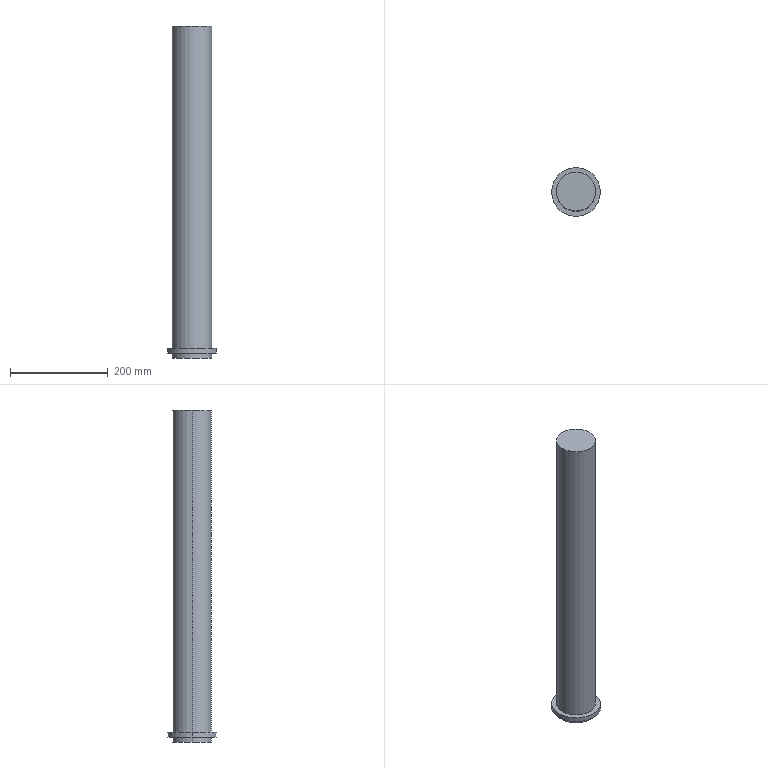Component | SolidWorks | ToolAxis-1 | 2 solids | 10 faces | box 100 x 100 x 680 mm | volume 3446327 mm3 | cylinder 6 | plane 4 | commonest cylinder face diameters 80 x4 100 x2
build123d program:
from build123d import *

# Parameters (mm, degrees)
SKETCH1_R           = 40
BOSS_EXTRUDE1_DEPTH = 680
BOSS_EXTRUDE2_START = -10
SKETCH2_R           = 50
SKETCH2_R_2         = 40
BOSS_EXTRUDE2_DEPTH = 10


with BuildPart() as part:
    # Sketch1 → Boss-Extrude1 (new body)
    with BuildSketch(Plane.XY):
        with Locations((0, -1000)):
            Circle(SKETCH1_R)
    extrude(amount=BOSS_EXTRUDE1_DEPTH)


with BuildPart() as body_2:
    # Sketch2 → Boss-Extrude2 (new body)
    with BuildSketch(Plane.XY.offset(680).offset(BOSS_EXTRUDE2_START)):
        with Locations((0, -1000)):
            Circle(SKETCH2_R)
        with Locations((0, -1000)):
            Circle(SKETCH2_R_2, mode=Mode.SUBTRACT)
    extrude(amount=-BOSS_EXTRUDE2_DEPTH)


solid = Compound([part.part, body_2.part])

# Placed as in the assembly
solid = solid.moved(Location((0, -2100, 110), (180, 0, 0)))
STEP:
#1=COLOUR_RGB('',0.7922,0.8196,0.9333);
#2=FILL_AREA_STYLE_COLOUR('',#1);
#3=FILL_AREA_STYLE('',(#2));
#4=SURFACE_STYLE_FILL_AREA(#3);
#5=SURFACE_SIDE_STYLE('',(#4));
#6=SURFACE_STYLE_USAGE(.BOTH.,#5);
#7=PRESENTATION_STYLE_ASSIGNMENT((#6));
#8=CARTESIAN_POINT('',(1.575,-43.307,-21.654));
#9=VERTEX_POINT('',#8);
#10=CARTESIAN_POINT('',(-1.575,-43.307,-21.654));
#11=VERTEX_POINT('',#10);
#12=CARTESIAN_POINT('',(-0.,-43.307,-21.654));
#13=DIRECTION('',(0.,0.,-1.));
#14=DIRECTION('',(-1.,0.,0.));
#15=AXIS2_PLACEMENT_3D('',#12,#13,#14);
#16=CIRCLE('',#15,1.575);
#17=EDGE_CURVE('',#9,#11,#16,.T.);
#18=ORIENTED_EDGE('',*,*,#17,.F.);
#19=CARTESIAN_POINT('',(1.575,-43.307,-22.047));
#20=VERTEX_POINT('',#19);
#21=CARTESIAN_POINT('',(1.575,-43.307,-21.654));
#22=DIRECTION('',(0.,0.,-1.));
#23=VECTOR('',#22,39.37);
#24=LINE('',#21,#23);
#25=EDGE_CURVE('',#9,#20,#24,.T.);
#26=ORIENTED_EDGE('',*,*,#25,.T.);
#27=CARTESIAN_POINT('',(-1.575,-43.307,-22.047));
#28=VERTEX_POINT('',#27);
#29=CARTESIAN_POINT('',(-0.,-43.307,-22.047));
#30=DIRECTION('',(0.,0.,-1.));
#31=DIRECTION('',(-1.,0.,0.));
#32=AXIS2_PLACEMENT_3D('',#29,#30,#31);
#33=CIRCLE('',#32,1.575);
#34=EDGE_CURVE('',#20,#28,#33,.T.);
#35=ORIENTED_EDGE('',*,*,#34,.T.);
#36=CARTESIAN_POINT('',(-1.575,-43.307,-21.654));
#37=DIRECTION('',(0.,0.,-1.));
#38=VECTOR('',#37,39.37);
#39=LINE('',#36,#38);
#40=EDGE_CURVE('',#11,#28,#39,.T.);
#41=ORIENTED_EDGE('',*,*,#40,.F.);
#42=EDGE_LOOP('',(#18,#26,#35,#41));
#43=FACE_OUTER_BOUND('',#42,.T.);
#44=CARTESIAN_POINT('',(-0.,-43.307,-21.654));
#45=DIRECTION('',(0.,0.,-1.));
#46=DIRECTION('',(-1.,0.,0.));
#47=AXIS2_PLACEMENT_3D('',#44,#45,#46);
#48=CYLINDRICAL_SURFACE('',#47,1.575);
#49=ADVANCED_FACE('',(#43),#48,.F.);
#50=CARTESIAN_POINT('',(-1.969,-43.307,-21.654));
#51=VERTEX_POINT('',#50);
#52=CARTESIAN_POINT('',(1.969,-43.307,-21.654));
#53=VERTEX_POINT('',#52);
#54=CARTESIAN_POINT('',(-0.,-43.307,-21.654));
#55=DIRECTION('',(0.,0.,-1.));
#56=DIRECTION('',(-1.,0.,0.));
#57=AXIS2_PLACEMENT_3D('',#54,#55,#56);
#58=CIRCLE('',#57,1.969);
#59=EDGE_CURVE('',#51,#53,#58,.T.);
#60=ORIENTED_EDGE('',*,*,#59,.T.);
#61=CARTESIAN_POINT('',(1.969,-43.307,-22.047));
#62=VERTEX_POINT('',#61);
#63=CARTESIAN_POINT('',(1.969,-43.307,-21.654));
#64=DIRECTION('',(0.,0.,-1.));
#65=VECTOR('',#64,39.37);
#66=LINE('',#63,#65);
#67=EDGE_CURVE('',#53,#62,#66,.T.);
#68=ORIENTED_EDGE('',*,*,#67,.T.);
#69=CARTESIAN_POINT('',(-1.969,-43.307,-22.047));
#70=VERTEX_POINT('',#69);
#71=CARTESIAN_POINT('',(-0.,-43.307,-22.047));
#72=DIRECTION('',(0.,0.,-1.));
#73=DIRECTION('',(-1.,0.,0.));
#74=AXIS2_PLACEMENT_3D('',#71,#72,#73);
#75=CIRCLE('',#74,1.969);
#76=EDGE_CURVE('',#70,#62,#75,.T.);
#77=ORIENTED_EDGE('',*,*,#76,.F.);
#78=CARTESIAN_POINT('',(-1.969,-43.307,-21.654));
#79=DIRECTION('',(0.,0.,-1.));
#80=VECTOR('',#79,39.37);
#81=LINE('',#78,#80);
#82=EDGE_CURVE('',#51,#70,#81,.T.);
#83=ORIENTED_EDGE('',*,*,#82,.F.);
#84=EDGE_LOOP('',(#60,#68,#77,#83));
#85=FACE_OUTER_BOUND('',#84,.T.);
#86=CARTESIAN_POINT('',(-0.,-43.307,-21.654));
#87=DIRECTION('',(0.,0.,-1.));
#88=DIRECTION('',(-1.,0.,0.));
#89=AXIS2_PLACEMENT_3D('',#86,#87,#88);
#90=CYLINDRICAL_SURFACE('',#89,1.969);
#91=ADVANCED_FACE('',(#85),#90,.T.);
#92=ORIENTED_EDGE('',*,*,#67,.F.);
#93=CARTESIAN_POINT('',(-0.,-43.307,-21.654));
#94=DIRECTION('',(0.,0.,-1.));
#95=DIRECTION('',(-1.,0.,0.));
#96=AXIS2_PLACEMENT_3D('',#93,#94,#95);
#97=CIRCLE('',#96,1.969);
#98=EDGE_CURVE('',#53,#51,#97,.T.);
#99=ORIENTED_EDGE('',*,*,#98,.T.);
#100=ORIENTED_EDGE('',*,*,#82,.T.);
#101=CARTESIAN_POINT('',(-0.,-43.307,-22.047));
#102=DIRECTION('',(0.,0.,-1.));
#103=DIRECTION('',(-1.,0.,0.));
#104=AXIS2_PLACEMENT_3D('',#101,#102,#103);
#105=CIRCLE('',#104,1.969);
#106=EDGE_CURVE('',#62,#70,#105,.T.);
#107=ORIENTED_EDGE('',*,*,#106,.F.);
#108=EDGE_LOOP('',(#92,#99,#100,#107));
#109=FACE_OUTER_BOUND('',#108,.T.);
#110=CARTESIAN_POINT('',(-0.,-43.307,-21.654));
#111=DIRECTION('',(0.,0.,-1.));
#112=DIRECTION('',(-1.,0.,0.));
#113=AXIS2_PLACEMENT_3D('',#110,#111,#112);
#114=CYLINDRICAL_SURFACE('',#113,1.969);
#115=ADVANCED_FACE('',(#109),#114,.T.);
#116=CARTESIAN_POINT('',(-0.,-43.307,-21.654));
#117=DIRECTION('',(0.,0.,-1.));
#118=DIRECTION('',(-1.,0.,0.));
#119=AXIS2_PLACEMENT_3D('',#116,#117,#118);
#120=CIRCLE('',#119,1.575);
#121=EDGE_CURVE('',#11,#9,#120,.T.);
#122=ORIENTED_EDGE('',*,*,#121,.T.);
#123=ORIENTED_EDGE('',*,*,#17,.T.);
#124=EDGE_LOOP('',(#122,#123));
#125=FACE_BOUND('',#124,.T.);
#126=ORIENTED_EDGE('',*,*,#59,.F.);
#127=ORIENTED_EDGE('',*,*,#98,.F.);
#128=EDGE_LOOP('',(#126,#127));
#129=FACE_OUTER_BOUND('',#128,.T.);
#130=CARTESIAN_POINT('',(-0.,-43.307,-21.654));
#131=DIRECTION('',(0.,0.,-1.));
#132=DIRECTION('',(-1.,0.,-0.));
#133=AXIS2_PLACEMENT_3D('',#130,#131,#132);
#134=PLANE('',#133);
#135=ADVANCED_FACE('',(#125,#129),#134,.F.);
#136=CARTESIAN_POINT('',(-0.,-43.307,-22.047));
#137=DIRECTION('',(0.,0.,-1.));
#138=DIRECTION('',(-1.,0.,0.));
#139=AXIS2_PLACEMENT_3D('',#136,#137,#138);
#140=CIRCLE('',#139,1.575);
#141=EDGE_CURVE('',#28,#20,#140,.T.);
#142=ORIENTED_EDGE('',*,*,#141,.F.);
#143=ORIENTED_EDGE('',*,*,#34,.F.);
#144=EDGE_LOOP('',(#142,#143));
#145=FACE_BOUND('',#144,.T.);
#146=ORIENTED_EDGE('',*,*,#76,.T.);
#147=ORIENTED_EDGE('',*,*,#106,.T.);
#148=EDGE_LOOP('',(#146,#147));
#149=FACE_OUTER_BOUND('',#148,.T.);
#150=CARTESIAN_POINT('',(-0.,-43.307,-22.047));
#151=DIRECTION('',(0.,0.,-1.));
#152=DIRECTION('',(-1.,0.,-0.));
#153=AXIS2_PLACEMENT_3D('',#150,#151,#152);
#154=PLANE('',#153);
#155=ADVANCED_FACE('',(#145,#149),#154,.T.);
#156=ORIENTED_EDGE('',*,*,#25,.F.);
#157=ORIENTED_EDGE('',*,*,#121,.F.);
#158=ORIENTED_EDGE('',*,*,#40,.T.);
#159=ORIENTED_EDGE('',*,*,#141,.T.);
#160=EDGE_LOOP('',(#156,#157,#158,#159));
#161=FACE_OUTER_BOUND('',#160,.T.);
#162=CARTESIAN_POINT('',(-0.,-43.307,-21.654));
#163=DIRECTION('',(0.,0.,-1.));
#164=DIRECTION('',(-1.,0.,0.));
#165=AXIS2_PLACEMENT_3D('',#162,#163,#164);
#166=CYLINDRICAL_SURFACE('',#165,1.575);
#167=ADVANCED_FACE('',(#161),#166,.F.);
#168=CLOSED_SHELL('',(#49,#91,#115,#135,#155,#167));
#169=MANIFOLD_SOLID_BREP('',#168);
#170=STYLED_ITEM('',(#7),#169);
#171=PRESENTATION_LAYER_ASSIGNMENT('','',(#170));
#172=COLOUR_RGB('',0.7922,0.8196,0.9333);
#173=FILL_AREA_STYLE_COLOUR('',#172);
#174=FILL_AREA_STYLE('',(#173));
#175=SURFACE_STYLE_FILL_AREA(#174);
#176=SURFACE_SIDE_STYLE('',(#175));
#177=SURFACE_STYLE_USAGE(.BOTH.,#176);
#178=PRESENTATION_STYLE_ASSIGNMENT((#177));
#179=CARTESIAN_POINT('',(-1.575,-43.307,-22.441));
#180=VERTEX_POINT('',#179);
#181=CARTESIAN_POINT('',(1.575,-43.307,-22.441));
#182=VERTEX_POINT('',#181);
#183=CARTESIAN_POINT('',(-0.,-43.307,-22.441));
#184=DIRECTION('',(0.,0.,-1.));
#185=DIRECTION('',(-1.,0.,0.));
#186=AXIS2_PLACEMENT_3D('',#183,#184,#185);
#187=CIRCLE('',#186,1.575);
#188=EDGE_CURVE('',#180,#182,#187,.T.);
#189=ORIENTED_EDGE('',*,*,#188,.F.);
#190=CARTESIAN_POINT('',(-1.575,-43.307,4.331));
#191=VERTEX_POINT('',#190);
#192=CARTESIAN_POINT('',(-1.575,-43.307,-22.441));
#193=DIRECTION('',(-0.,-0.,1.));
#194=VECTOR('',#193,39.37);
#195=LINE('',#192,#194);
#196=EDGE_CURVE('',#180,#191,#195,.T.);
#197=ORIENTED_EDGE('',*,*,#196,.T.);
#198=CARTESIAN_POINT('',(1.575,-43.307,4.331));
#199=VERTEX_POINT('',#198);
#200=CARTESIAN_POINT('',(-0.,-43.307,4.331));
#201=DIRECTION('',(0.,0.,-1.));
#202=DIRECTION('',(-1.,0.,0.));
#203=AXIS2_PLACEMENT_3D('',#200,#201,#202);
#204=CIRCLE('',#203,1.575);
#205=EDGE_CURVE('',#191,#199,#204,.T.);
#206=ORIENTED_EDGE('',*,*,#205,.T.);
#207=CARTESIAN_POINT('',(1.575,-43.307,-22.441));
#208=DIRECTION('',(-0.,-0.,1.));
#209=VECTOR('',#208,39.37);
#210=LINE('',#207,#209);
#211=EDGE_CURVE('',#182,#199,#210,.T.);
#212=ORIENTED_EDGE('',*,*,#211,.F.);
#213=EDGE_LOOP('',(#189,#197,#206,#212));
#214=FACE_OUTER_BOUND('',#213,.T.);
#215=CARTESIAN_POINT('',(-0.,-43.307,-22.441));
#216=DIRECTION('',(-0.,-0.,1.));
#217=DIRECTION('',(1.,0.,0.));
#218=AXIS2_PLACEMENT_3D('',#215,#216,#217);
#219=CYLINDRICAL_SURFACE('',#218,1.575);
#220=ADVANCED_FACE('',(#214),#219,.T.);
#221=ORIENTED_EDGE('',*,*,#196,.F.);
#222=CARTESIAN_POINT('',(-0.,-43.307,-22.441));
#223=DIRECTION('',(0.,0.,-1.));
#224=DIRECTION('',(-1.,0.,0.));
#225=AXIS2_PLACEMENT_3D('',#222,#223,#224);
#226=CIRCLE('',#225,1.575);
#227=EDGE_CURVE('',#182,#180,#226,.T.);
#228=ORIENTED_EDGE('',*,*,#227,.F.);
#229=ORIENTED_EDGE('',*,*,#211,.T.);
#230=CARTESIAN_POINT('',(-0.,-43.307,4.331));
#231=DIRECTION('',(0.,0.,-1.));
#232=DIRECTION('',(-1.,0.,0.));
#233=AXIS2_PLACEMENT_3D('',#230,#231,#232);
#234=CIRCLE('',#233,1.575);
#235=EDGE_CURVE('',#199,#191,#234,.T.);
#236=ORIENTED_EDGE('',*,*,#235,.T.);
#237=EDGE_LOOP('',(#221,#228,#229,#236));
#238=FACE_OUTER_BOUND('',#237,.T.);
#239=CARTESIAN_POINT('',(-0.,-43.307,-22.441));
#240=DIRECTION('',(-0.,-0.,1.));
#241=DIRECTION('',(1.,0.,0.));
#242=AXIS2_PLACEMENT_3D('',#239,#240,#241);
#243=CYLINDRICAL_SURFACE('',#242,1.575);
#244=ADVANCED_FACE('',(#238),#243,.T.);
#245=ORIENTED_EDGE('',*,*,#227,.T.);
#246=ORIENTED_EDGE('',*,*,#188,.T.);
#247=EDGE_LOOP('',(#245,#246));
#248=FACE_OUTER_BOUND('',#247,.T.);
#249=CARTESIAN_POINT('',(-0.,-43.307,-22.441));
#250=DIRECTION('',(0.,0.,-1.));
#251=DIRECTION('',(-1.,0.,-0.));
#252=AXIS2_PLACEMENT_3D('',#249,#250,#251);
#253=PLANE('',#252);
#254=ADVANCED_FACE('',(#248),#253,.T.);
#255=ORIENTED_EDGE('',*,*,#235,.F.);
#256=ORIENTED_EDGE('',*,*,#205,.F.);
#257=EDGE_LOOP('',(#255,#256));
#258=FACE_OUTER_BOUND('',#257,.T.);
#259=CARTESIAN_POINT('',(-0.,-43.307,4.331));
#260=DIRECTION('',(0.,0.,-1.));
#261=DIRECTION('',(-1.,0.,-0.));
#262=AXIS2_PLACEMENT_3D('',#259,#260,#261);
#263=PLANE('',#262);
#264=ADVANCED_FACE('',(#258),#263,.F.);
#265=CLOSED_SHELL('',(#220,#244,#254,#264));
#266=MANIFOLD_SOLID_BREP('',#265);
#267=STYLED_ITEM('',(#178),#266);
#268=PRESENTATION_LAYER_ASSIGNMENT('','',(#267));
#269=CARTESIAN_POINT('',(0.,0.,0.));
#270=DIRECTION('',(0.,0.,1.));
#271=DIRECTION('',(1.,0.,0.));
#272=AXIS2_PLACEMENT_3D('',#269,#270,#271);
#273=(LENGTH_UNIT()NAMED_UNIT(*)SI_UNIT($,.METRE.));
#274=LENGTH_MEASURE_WITH_UNIT(LENGTH_MEASURE(0.0254),#273);
#275=DIMENSIONAL_EXPONENTS(1.,0.,0.,0.,0.,0.,0.);
#276=(CONVERSION_BASED_UNIT('',#274)LENGTH_UNIT()NAMED_UNIT(#275));
#277=UNCERTAINTY_MEASURE_WITH_UNIT(LENGTH_MEASURE(0.00001),#276,'','');
#278=(NAMED_UNIT(*)PLANE_ANGLE_UNIT()SI_UNIT($,.RADIAN.));
#279=(NAMED_UNIT(*)SI_UNIT($,.STERADIAN.)SOLID_ANGLE_UNIT());
#280=(GEOMETRIC_REPRESENTATION_CONTEXT(3)GLOBAL_UNCERTAINTY_ASSIGNED_CONTEXT((#277))GLOBAL_UNIT_ASSIGNED_CONTEXT((#276,#278,#279))REPRESENTATION_CONTEXT('',''));
#281=ADVANCED_BREP_SHAPE_REPRESENTATION('',(#169,#266,#272),#280);
#282=(LENGTH_UNIT()NAMED_UNIT(*)SI_UNIT($,.METRE.));
#283=LENGTH_MEASURE_WITH_UNIT(LENGTH_MEASURE(0.0254),#282);
#284=DIMENSIONAL_EXPONENTS(1.,0.,0.,0.,0.,0.,0.);
#285=(CONVERSION_BASED_UNIT('',#283)LENGTH_UNIT()NAMED_UNIT(#284));
#286=UNCERTAINTY_MEASURE_WITH_UNIT(LENGTH_MEASURE(0.00001),#285,'','');
#287=(NAMED_UNIT(*)PLANE_ANGLE_UNIT()SI_UNIT($,.RADIAN.));
#288=(NAMED_UNIT(*)SI_UNIT($,.STERADIAN.)SOLID_ANGLE_UNIT());
#289=(GEOMETRIC_REPRESENTATION_CONTEXT(3)GLOBAL_UNCERTAINTY_ASSIGNED_CONTEXT((#286))GLOBAL_UNIT_ASSIGNED_CONTEXT((#285,#287,#288))REPRESENTATION_CONTEXT('',''));
#290=MECHANICAL_DESIGN_GEOMETRIC_PRESENTATION_REPRESENTATION('',(#170),#289);
#291=(LENGTH_UNIT()NAMED_UNIT(*)SI_UNIT($,.METRE.));
#292=LENGTH_MEASURE_WITH_UNIT(LENGTH_MEASURE(0.0254),#291);
#293=DIMENSIONAL_EXPONENTS(1.,0.,0.,0.,0.,0.,0.);
#294=(CONVERSION_BASED_UNIT('',#292)LENGTH_UNIT()NAMED_UNIT(#293));
#295=UNCERTAINTY_MEASURE_WITH_UNIT(LENGTH_MEASURE(0.00001),#294,'','');
#296=(NAMED_UNIT(*)PLANE_ANGLE_UNIT()SI_UNIT($,.RADIAN.));
#297=(NAMED_UNIT(*)SI_UNIT($,.STERADIAN.)SOLID_ANGLE_UNIT());
#298=(GEOMETRIC_REPRESENTATION_CONTEXT(3)GLOBAL_UNCERTAINTY_ASSIGNED_CONTEXT((#295))GLOBAL_UNIT_ASSIGNED_CONTEXT((#294,#296,#297))REPRESENTATION_CONTEXT('',''));
#299=MECHANICAL_DESIGN_GEOMETRIC_PRESENTATION_REPRESENTATION('',(#267),#298);